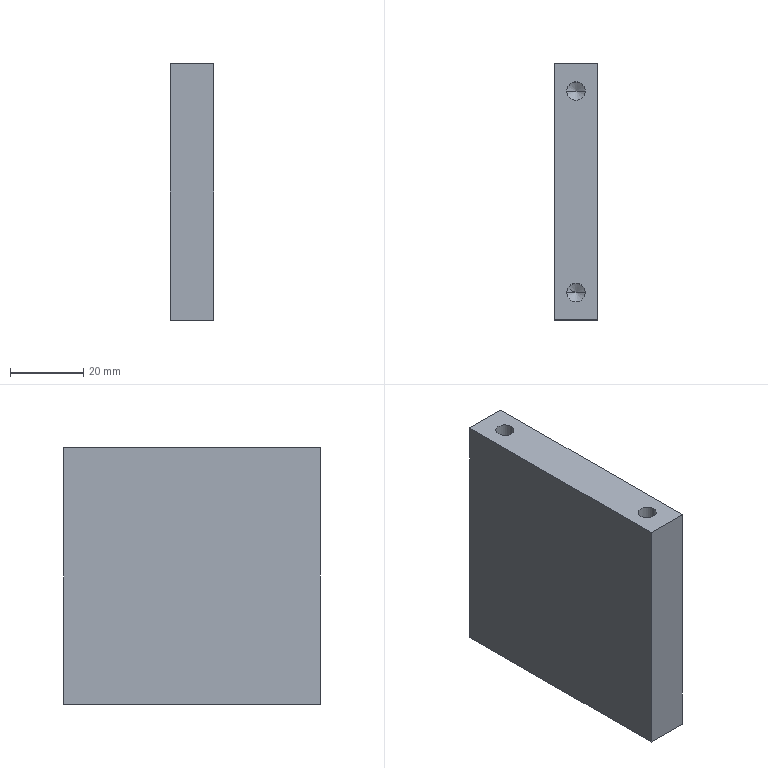Component | SolidWorks | ServoDriveMotorModule-1_WT-FLD-EJG-1212-00-020-1 | 1 solid | 22 faces | box 12 x 70 x 70 mm | volume 57583 mm3 | cylinder 8 | cone 8 | plane 6 | commonest cylinder face diameters 5 x8 | material AISI 1045 Steel, cold drawn
build123d program:
from build123d import *

# Parameters (mm, degrees)
SKETCH1_W                  = 12
SKETCH1_H                  = 70
BOSS_EXTRUDE1_DEPTH        = 35
M6_TAPPED_HOLE1_AT_2_COUNT = 2
M6_TAPPED_HOLE1_AT_2_PITCH = 55


with BuildPart() as part:
    # Sketch1 → Boss-Extrude1 (new, symmetric)
    with BuildSketch(Plane.XY):
        Rectangle(SKETCH1_W, SKETCH1_H)
    extrude(amount=BOSS_EXTRUDE1_DEPTH, both=True)

    # Sketch2 → M6 Tapped Hole1 (revolve, cut)
    with BuildSketch(Plane(origin=(0, 27.5, 35), x_dir=(0, -1, 0), z_dir=(1, 0, 0))):
        Polygon((0, 0), (0, 16.502), (2.5, 15), (2.5, 0), align=None)
    m6_tapped_hole1 = revolve(axis=Axis((0, 27.5, 41.35), (0, 0, -1)), mode=Mode.SUBTRACT)

    # M6 Tapped Hole1 at 2: M6 Tapped Hole1 ×2
    with Locations(*[(0, -i * M6_TAPPED_HOLE1_AT_2_PITCH, 0) for i in range(1, M6_TAPPED_HOLE1_AT_2_COUNT)]):
        add(m6_tapped_hole1, mode=Mode.SUBTRACT)

    # Mirror1: M6 Tapped Hole1 across plane
    add(m6_tapped_hole1.mirror(Plane.XY), mode=Mode.SUBTRACT)

    # Mirror1 copy 1 sketch → Mirror1 copy 1 (revolve, cut)
    with BuildSketch(Plane(origin=(0, -27.5, -35), x_dir=(0, -1, 0), z_dir=(1, 0, 0))):
        Polygon((0, 0), (0, -16.502), (2.5, -15), (2.5, 0), align=None)
    revolve(axis=Axis((0, -27.5, -41.35), (0, 0, -1)), mode=Mode.SUBTRACT)


solid = part.part

# Placed as in the assembly
solid = solid.moved(Location((-49, 0, 95), (0, 0, 0)))
STEP:
#1=CARTESIAN_POINT('',(-2.028,1.083,4.528));
#2=VERTEX_POINT('',#1);
#3=CARTESIAN_POINT('',(-1.831,1.083,4.528));
#4=VERTEX_POINT('',#3);
#5=CARTESIAN_POINT('',(-1.929,1.083,4.528));
#6=DIRECTION('',(0.,-0.,1.));
#7=DIRECTION('',(1.,0.,0.));
#8=AXIS2_PLACEMENT_3D('',#5,#6,#7);
#9=CIRCLE('',#8,0.09843);
#10=EDGE_CURVE('',#2,#4,#9,.T.);
#11=ORIENTED_EDGE('',*,*,#10,.F.);
#12=CARTESIAN_POINT('',(-2.028,1.083,5.118));
#13=VERTEX_POINT('',#12);
#14=CARTESIAN_POINT('',(-2.028,1.083,5.118));
#15=DIRECTION('',(0.,-0.,1.));
#16=VECTOR('',#15,39.37);
#17=LINE('',#14,#16);
#18=EDGE_CURVE('',#2,#13,#17,.T.);
#19=ORIENTED_EDGE('',*,*,#18,.T.);
#20=CARTESIAN_POINT('',(-1.831,1.083,5.118));
#21=VERTEX_POINT('',#20);
#22=CARTESIAN_POINT('',(-1.929,1.083,5.118));
#23=DIRECTION('',(0.,-0.,1.));
#24=DIRECTION('',(1.,0.,0.));
#25=AXIS2_PLACEMENT_3D('',#22,#23,#24);
#26=CIRCLE('',#25,0.09843);
#27=EDGE_CURVE('',#13,#21,#26,.T.);
#28=ORIENTED_EDGE('',*,*,#27,.T.);
#29=CARTESIAN_POINT('',(-1.831,1.083,5.118));
#30=DIRECTION('',(0.,-0.,1.));
#31=VECTOR('',#30,39.37);
#32=LINE('',#29,#31);
#33=EDGE_CURVE('',#4,#21,#32,.T.);
#34=ORIENTED_EDGE('',*,*,#33,.F.);
#35=EDGE_LOOP('',(#11,#19,#28,#34));
#36=FACE_OUTER_BOUND('',#35,.T.);
#37=CARTESIAN_POINT('',(-1.929,1.083,5.118));
#38=DIRECTION('',(0.,-0.,1.));
#39=DIRECTION('',(1.,0.,0.));
#40=AXIS2_PLACEMENT_3D('',#37,#38,#39);
#41=CYLINDRICAL_SURFACE('',#40,0.09843);
#42=ADVANCED_FACE('',(#36),#41,.F.);
#43=CARTESIAN_POINT('',(-1.929,1.083,4.468));
#44=VERTEX_POINT('',#43);
#45=CARTESIAN_POINT('',(-1.831,1.083,4.528));
#46=DIRECTION('',(0.8572,0.,0.515));
#47=VECTOR('',#46,39.37);
#48=LINE('',#45,#47);
#49=EDGE_CURVE('',#44,#4,#48,.T.);
#50=ORIENTED_EDGE('',*,*,#49,.F.);
#51=CARTESIAN_POINT('',(-2.028,1.083,4.528));
#52=DIRECTION('',(-0.8572,-0.,0.515));
#53=VECTOR('',#52,39.37);
#54=LINE('',#51,#53);
#55=EDGE_CURVE('',#44,#2,#54,.T.);
#56=ORIENTED_EDGE('',*,*,#55,.T.);
#57=ORIENTED_EDGE('',*,*,#10,.T.);
#58=EDGE_LOOP('',(#50,#56,#57));
#59=FACE_OUTER_BOUND('',#58,.T.);
#60=CARTESIAN_POINT('',(-1.929,1.083,4.528));
#61=DIRECTION('',(0.,-0.,1.));
#62=DIRECTION('',(1.,0.,0.));
#63=AXIS2_PLACEMENT_3D('',#60,#61,#62);
#64=CONICAL_SURFACE('',#63,0.09843,1.03);
#65=ADVANCED_FACE('',(#59),#64,.F.);
#66=CARTESIAN_POINT('',(-2.028,-1.083,4.528));
#67=VERTEX_POINT('',#66);
#68=CARTESIAN_POINT('',(-1.831,-1.083,4.528));
#69=VERTEX_POINT('',#68);
#70=CARTESIAN_POINT('',(-1.929,-1.083,4.528));
#71=DIRECTION('',(0.,-0.,1.));
#72=DIRECTION('',(1.,0.,0.));
#73=AXIS2_PLACEMENT_3D('',#70,#71,#72);
#74=CIRCLE('',#73,0.09843);
#75=EDGE_CURVE('',#67,#69,#74,.T.);
#76=ORIENTED_EDGE('',*,*,#75,.F.);
#77=CARTESIAN_POINT('',(-2.028,-1.083,5.118));
#78=VERTEX_POINT('',#77);
#79=CARTESIAN_POINT('',(-2.028,-1.083,5.118));
#80=DIRECTION('',(0.,-0.,1.));
#81=VECTOR('',#80,39.37);
#82=LINE('',#79,#81);
#83=EDGE_CURVE('',#67,#78,#82,.T.);
#84=ORIENTED_EDGE('',*,*,#83,.T.);
#85=CARTESIAN_POINT('',(-1.831,-1.083,5.118));
#86=VERTEX_POINT('',#85);
#87=CARTESIAN_POINT('',(-1.929,-1.083,5.118));
#88=DIRECTION('',(0.,-0.,1.));
#89=DIRECTION('',(1.,0.,0.));
#90=AXIS2_PLACEMENT_3D('',#87,#88,#89);
#91=CIRCLE('',#90,0.09843);
#92=EDGE_CURVE('',#78,#86,#91,.T.);
#93=ORIENTED_EDGE('',*,*,#92,.T.);
#94=CARTESIAN_POINT('',(-1.831,-1.083,5.118));
#95=DIRECTION('',(0.,-0.,1.));
#96=VECTOR('',#95,39.37);
#97=LINE('',#94,#96);
#98=EDGE_CURVE('',#69,#86,#97,.T.);
#99=ORIENTED_EDGE('',*,*,#98,.F.);
#100=EDGE_LOOP('',(#76,#84,#93,#99));
#101=FACE_OUTER_BOUND('',#100,.T.);
#102=CARTESIAN_POINT('',(-1.929,-1.083,5.118));
#103=DIRECTION('',(0.,-0.,1.));
#104=DIRECTION('',(1.,0.,0.));
#105=AXIS2_PLACEMENT_3D('',#102,#103,#104);
#106=CYLINDRICAL_SURFACE('',#105,0.09843);
#107=ADVANCED_FACE('',(#101),#106,.F.);
#108=CARTESIAN_POINT('',(-1.929,-1.083,4.468));
#109=VERTEX_POINT('',#108);
#110=CARTESIAN_POINT('',(-1.831,-1.083,4.528));
#111=DIRECTION('',(0.8572,0.,0.515));
#112=VECTOR('',#111,39.37);
#113=LINE('',#110,#112);
#114=EDGE_CURVE('',#109,#69,#113,.T.);
#115=ORIENTED_EDGE('',*,*,#114,.F.);
#116=CARTESIAN_POINT('',(-2.028,-1.083,4.528));
#117=DIRECTION('',(-0.8572,-0.,0.515));
#118=VECTOR('',#117,39.37);
#119=LINE('',#116,#118);
#120=EDGE_CURVE('',#109,#67,#119,.T.);
#121=ORIENTED_EDGE('',*,*,#120,.T.);
#122=ORIENTED_EDGE('',*,*,#75,.T.);
#123=EDGE_LOOP('',(#115,#121,#122));
#124=FACE_OUTER_BOUND('',#123,.T.);
#125=CARTESIAN_POINT('',(-1.929,-1.083,4.528));
#126=DIRECTION('',(0.,-0.,1.));
#127=DIRECTION('',(1.,0.,0.));
#128=AXIS2_PLACEMENT_3D('',#125,#126,#127);
#129=CONICAL_SURFACE('',#128,0.09843,1.03);
#130=ADVANCED_FACE('',(#124),#129,.F.);
#131=CARTESIAN_POINT('',(-1.831,1.083,2.953));
#132=VERTEX_POINT('',#131);
#133=CARTESIAN_POINT('',(-2.028,1.083,2.953));
#134=VERTEX_POINT('',#133);
#135=CARTESIAN_POINT('',(-1.929,1.083,2.953));
#136=DIRECTION('',(-0.,0.,-1.));
#137=DIRECTION('',(-1.,-0.,0.));
#138=AXIS2_PLACEMENT_3D('',#135,#136,#137);
#139=CIRCLE('',#138,0.09843);
#140=EDGE_CURVE('',#132,#134,#139,.T.);
#141=ORIENTED_EDGE('',*,*,#140,.F.);
#142=CARTESIAN_POINT('',(-1.831,1.083,2.362));
#143=VERTEX_POINT('',#142);
#144=CARTESIAN_POINT('',(-1.831,1.083,2.362));
#145=DIRECTION('',(-0.,0.,-1.));
#146=VECTOR('',#145,39.37);
#147=LINE('',#144,#146);
#148=EDGE_CURVE('',#132,#143,#147,.T.);
#149=ORIENTED_EDGE('',*,*,#148,.T.);
#150=CARTESIAN_POINT('',(-2.028,1.083,2.362));
#151=VERTEX_POINT('',#150);
#152=CARTESIAN_POINT('',(-1.929,1.083,2.362));
#153=DIRECTION('',(-0.,0.,-1.));
#154=DIRECTION('',(-1.,-0.,0.));
#155=AXIS2_PLACEMENT_3D('',#152,#153,#154);
#156=CIRCLE('',#155,0.09843);
#157=EDGE_CURVE('',#143,#151,#156,.T.);
#158=ORIENTED_EDGE('',*,*,#157,.T.);
#159=CARTESIAN_POINT('',(-2.028,1.083,2.362));
#160=DIRECTION('',(-0.,0.,-1.));
#161=VECTOR('',#160,39.37);
#162=LINE('',#159,#161);
#163=EDGE_CURVE('',#134,#151,#162,.T.);
#164=ORIENTED_EDGE('',*,*,#163,.F.);
#165=EDGE_LOOP('',(#141,#149,#158,#164));
#166=FACE_OUTER_BOUND('',#165,.T.);
#167=CARTESIAN_POINT('',(-1.929,1.083,2.362));
#168=DIRECTION('',(-0.,0.,-1.));
#169=DIRECTION('',(-1.,-0.,0.));
#170=AXIS2_PLACEMENT_3D('',#167,#168,#169);
#171=CYLINDRICAL_SURFACE('',#170,0.09843);
#172=ADVANCED_FACE('',(#166),#171,.F.);
#173=CARTESIAN_POINT('',(-1.929,1.083,3.012));
#174=VERTEX_POINT('',#173);
#175=CARTESIAN_POINT('',(-2.028,1.083,2.953));
#176=DIRECTION('',(-0.8572,-0.,-0.515));
#177=VECTOR('',#176,39.37);
#178=LINE('',#175,#177);
#179=EDGE_CURVE('',#174,#134,#178,.T.);
#180=ORIENTED_EDGE('',*,*,#179,.F.);
#181=CARTESIAN_POINT('',(-1.831,1.083,2.953));
#182=DIRECTION('',(0.8572,0.,-0.515));
#183=VECTOR('',#182,39.37);
#184=LINE('',#181,#183);
#185=EDGE_CURVE('',#174,#132,#184,.T.);
#186=ORIENTED_EDGE('',*,*,#185,.T.);
#187=ORIENTED_EDGE('',*,*,#140,.T.);
#188=EDGE_LOOP('',(#180,#186,#187));
#189=FACE_OUTER_BOUND('',#188,.T.);
#190=CARTESIAN_POINT('',(-1.929,1.083,2.953));
#191=DIRECTION('',(-0.,0.,-1.));
#192=DIRECTION('',(-1.,-0.,0.));
#193=AXIS2_PLACEMENT_3D('',#190,#191,#192);
#194=CONICAL_SURFACE('',#193,0.09843,1.03);
#195=ADVANCED_FACE('',(#189),#194,.F.);
#196=CARTESIAN_POINT('',(-1.831,-1.083,2.953));
#197=VERTEX_POINT('',#196);
#198=CARTESIAN_POINT('',(-2.028,-1.083,2.953));
#199=VERTEX_POINT('',#198);
#200=CARTESIAN_POINT('',(-1.929,-1.083,2.953));
#201=DIRECTION('',(-0.,0.,-1.));
#202=DIRECTION('',(-1.,-0.,0.));
#203=AXIS2_PLACEMENT_3D('',#200,#201,#202);
#204=CIRCLE('',#203,0.09843);
#205=EDGE_CURVE('',#197,#199,#204,.T.);
#206=ORIENTED_EDGE('',*,*,#205,.F.);
#207=CARTESIAN_POINT('',(-1.831,-1.083,2.362));
#208=VERTEX_POINT('',#207);
#209=CARTESIAN_POINT('',(-1.831,-1.083,2.362));
#210=DIRECTION('',(-0.,0.,-1.));
#211=VECTOR('',#210,39.37);
#212=LINE('',#209,#211);
#213=EDGE_CURVE('',#197,#208,#212,.T.);
#214=ORIENTED_EDGE('',*,*,#213,.T.);
#215=CARTESIAN_POINT('',(-2.028,-1.083,2.362));
#216=VERTEX_POINT('',#215);
#217=CARTESIAN_POINT('',(-1.929,-1.083,2.362));
#218=DIRECTION('',(-0.,0.,-1.));
#219=DIRECTION('',(-1.,-0.,0.));
#220=AXIS2_PLACEMENT_3D('',#217,#218,#219);
#221=CIRCLE('',#220,0.09843);
#222=EDGE_CURVE('',#208,#216,#221,.T.);
#223=ORIENTED_EDGE('',*,*,#222,.T.);
#224=CARTESIAN_POINT('',(-2.028,-1.083,2.362));
#225=DIRECTION('',(-0.,0.,-1.));
#226=VECTOR('',#225,39.37);
#227=LINE('',#224,#226);
#228=EDGE_CURVE('',#199,#216,#227,.T.);
#229=ORIENTED_EDGE('',*,*,#228,.F.);
#230=EDGE_LOOP('',(#206,#214,#223,#229));
#231=FACE_OUTER_BOUND('',#230,.T.);
#232=CARTESIAN_POINT('',(-1.929,-1.083,2.362));
#233=DIRECTION('',(-0.,0.,-1.));
#234=DIRECTION('',(-1.,-0.,0.));
#235=AXIS2_PLACEMENT_3D('',#232,#233,#234);
#236=CYLINDRICAL_SURFACE('',#235,0.09843);
#237=ADVANCED_FACE('',(#231),#236,.F.);
#238=CARTESIAN_POINT('',(-1.929,-1.083,3.012));
#239=VERTEX_POINT('',#238);
#240=CARTESIAN_POINT('',(-2.028,-1.083,2.953));
#241=DIRECTION('',(-0.8572,-0.,-0.515));
#242=VECTOR('',#241,39.37);
#243=LINE('',#240,#242);
#244=EDGE_CURVE('',#239,#199,#243,.T.);
#245=ORIENTED_EDGE('',*,*,#244,.F.);
#246=CARTESIAN_POINT('',(-1.831,-1.083,2.953));
#247=DIRECTION('',(0.8572,0.,-0.515));
#248=VECTOR('',#247,39.37);
#249=LINE('',#246,#248);
#250=EDGE_CURVE('',#239,#197,#249,.T.);
#251=ORIENTED_EDGE('',*,*,#250,.T.);
#252=ORIENTED_EDGE('',*,*,#205,.T.);
#253=EDGE_LOOP('',(#245,#251,#252));
#254=FACE_OUTER_BOUND('',#253,.T.);
#255=CARTESIAN_POINT('',(-1.929,-1.083,2.953));
#256=DIRECTION('',(-0.,0.,-1.));
#257=DIRECTION('',(-1.,-0.,0.));
#258=AXIS2_PLACEMENT_3D('',#255,#256,#257);
#259=CONICAL_SURFACE('',#258,0.09843,1.03);
#260=ADVANCED_FACE('',(#254),#259,.F.);
#261=CARTESIAN_POINT('',(-2.165,-1.378,5.118));
#262=VERTEX_POINT('',#261);
#263=CARTESIAN_POINT('',(-2.165,1.378,5.118));
#264=VERTEX_POINT('',#263);
#265=CARTESIAN_POINT('',(-2.165,-1.378,5.118));
#266=DIRECTION('',(-0.,1.,0.));
#267=VECTOR('',#266,39.37);
#268=LINE('',#265,#267);
#269=EDGE_CURVE('',#262,#264,#268,.T.);
#270=ORIENTED_EDGE('',*,*,#269,.T.);
#271=CARTESIAN_POINT('',(-2.165,1.378,2.362));
#272=VERTEX_POINT('',#271);
#273=CARTESIAN_POINT('',(-2.165,1.378,2.362));
#274=DIRECTION('',(0.,-0.,1.));
#275=VECTOR('',#274,39.37);
#276=LINE('',#273,#275);
#277=EDGE_CURVE('',#272,#264,#276,.T.);
#278=ORIENTED_EDGE('',*,*,#277,.F.);
#279=CARTESIAN_POINT('',(-2.165,-1.378,2.362));
#280=VERTEX_POINT('',#279);
#281=CARTESIAN_POINT('',(-2.165,-1.378,2.362));
#282=DIRECTION('',(-0.,1.,0.));
#283=VECTOR('',#282,39.37);
#284=LINE('',#281,#283);
#285=EDGE_CURVE('',#280,#272,#284,.T.);
#286=ORIENTED_EDGE('',*,*,#285,.F.);
#287=CARTESIAN_POINT('',(-2.165,-1.378,2.362));
#288=DIRECTION('',(0.,-0.,1.));
#289=VECTOR('',#288,39.37);
#290=LINE('',#287,#289);
#291=EDGE_CURVE('',#280,#262,#290,.T.);
#292=ORIENTED_EDGE('',*,*,#291,.T.);
#293=EDGE_LOOP('',(#270,#278,#286,#292));
#294=FACE_OUTER_BOUND('',#293,.T.);
#295=CARTESIAN_POINT('',(-2.165,-1.378,2.362));
#296=DIRECTION('',(1.,0.,-0.));
#297=DIRECTION('',(-0.,0.,-1.));
#298=AXIS2_PLACEMENT_3D('',#295,#296,#297);
#299=PLANE('',#298);
#300=ADVANCED_FACE('',(#294),#299,.F.);
#301=CARTESIAN_POINT('',(-1.693,1.378,5.118));
#302=VERTEX_POINT('',#301);
#303=CARTESIAN_POINT('',(-1.693,1.378,5.118));
#304=DIRECTION('',(1.,0.,-0.));
#305=VECTOR('',#304,39.37);
#306=LINE('',#303,#305);
#307=EDGE_CURVE('',#264,#302,#306,.T.);
#308=ORIENTED_EDGE('',*,*,#307,.T.);
#309=CARTESIAN_POINT('',(-1.693,1.378,2.362));
#310=VERTEX_POINT('',#309);
#311=CARTESIAN_POINT('',(-1.693,1.378,2.362));
#312=DIRECTION('',(0.,-0.,1.));
#313=VECTOR('',#312,39.37);
#314=LINE('',#311,#313);
#315=EDGE_CURVE('',#310,#302,#314,.T.);
#316=ORIENTED_EDGE('',*,*,#315,.F.);
#317=CARTESIAN_POINT('',(-1.693,1.378,2.362));
#318=DIRECTION('',(1.,0.,-0.));
#319=VECTOR('',#318,39.37);
#320=LINE('',#317,#319);
#321=EDGE_CURVE('',#272,#310,#320,.T.);
#322=ORIENTED_EDGE('',*,*,#321,.F.);
#323=ORIENTED_EDGE('',*,*,#277,.T.);
#324=EDGE_LOOP('',(#308,#316,#322,#323));
#325=FACE_OUTER_BOUND('',#324,.T.);
#326=CARTESIAN_POINT('',(-1.693,1.378,2.362));
#327=DIRECTION('',(0.,-1.,-0.));
#328=DIRECTION('',(0.,-0.,1.));
#329=AXIS2_PLACEMENT_3D('',#326,#327,#328);
#330=PLANE('',#329);
#331=ADVANCED_FACE('',(#325),#330,.F.);
#332=CARTESIAN_POINT('',(-1.693,-1.378,5.118));
#333=VERTEX_POINT('',#332);
#334=CARTESIAN_POINT('',(-1.693,-1.378,5.118));
#335=DIRECTION('',(0.,-1.,-0.));
#336=VECTOR('',#335,39.37);
#337=LINE('',#334,#336);
#338=EDGE_CURVE('',#302,#333,#337,.T.);
#339=ORIENTED_EDGE('',*,*,#338,.T.);
#340=CARTESIAN_POINT('',(-1.693,-1.378,2.362));
#341=VERTEX_POINT('',#340);
#342=CARTESIAN_POINT('',(-1.693,-1.378,2.362));
#343=DIRECTION('',(0.,-0.,1.));
#344=VECTOR('',#343,39.37);
#345=LINE('',#342,#344);
#346=EDGE_CURVE('',#341,#333,#345,.T.);
#347=ORIENTED_EDGE('',*,*,#346,.F.);
#348=CARTESIAN_POINT('',(-1.693,-1.378,2.362));
#349=DIRECTION('',(0.,-1.,-0.));
#350=VECTOR('',#349,39.37);
#351=LINE('',#348,#350);
#352=EDGE_CURVE('',#310,#341,#351,.T.);
#353=ORIENTED_EDGE('',*,*,#352,.F.);
#354=ORIENTED_EDGE('',*,*,#315,.T.);
#355=EDGE_LOOP('',(#339,#347,#353,#354));
#356=FACE_OUTER_BOUND('',#355,.T.);
#357=CARTESIAN_POINT('',(-1.693,-1.378,2.362));
#358=DIRECTION('',(-1.,-0.,0.));
#359=DIRECTION('',(0.,-0.,1.));
#360=AXIS2_PLACEMENT_3D('',#357,#358,#359);
#361=PLANE('',#360);
#362=ADVANCED_FACE('',(#356),#361,.F.);
#363=CARTESIAN_POINT('',(-1.693,-1.378,5.118));
#364=DIRECTION('',(-1.,-0.,0.));
#365=VECTOR('',#364,39.37);
#366=LINE('',#363,#365);
#367=EDGE_CURVE('',#333,#262,#366,.T.);
#368=ORIENTED_EDGE('',*,*,#367,.T.);
#369=ORIENTED_EDGE('',*,*,#291,.F.);
#370=CARTESIAN_POINT('',(-1.693,-1.378,2.362));
#371=DIRECTION('',(-1.,-0.,0.));
#372=VECTOR('',#371,39.37);
#373=LINE('',#370,#372);
#374=EDGE_CURVE('',#341,#280,#373,.T.);
#375=ORIENTED_EDGE('',*,*,#374,.F.);
#376=ORIENTED_EDGE('',*,*,#346,.T.);
#377=EDGE_LOOP('',(#368,#369,#375,#376));
#378=FACE_OUTER_BOUND('',#377,.T.);
#379=CARTESIAN_POINT('',(-1.693,-1.378,2.362));
#380=DIRECTION('',(-0.,1.,0.));
#381=DIRECTION('',(-0.,0.,-1.));
#382=AXIS2_PLACEMENT_3D('',#379,#380,#381);
#383=PLANE('',#382);
#384=ADVANCED_FACE('',(#378),#383,.F.);
#385=CARTESIAN_POINT('',(-1.929,1.083,2.362));
#386=DIRECTION('',(-0.,0.,-1.));
#387=DIRECTION('',(-1.,-0.,0.));
#388=AXIS2_PLACEMENT_3D('',#385,#386,#387);
#389=CIRCLE('',#388,0.09843);
#390=EDGE_CURVE('',#151,#143,#389,.T.);
#391=ORIENTED_EDGE('',*,*,#390,.F.);
#392=ORIENTED_EDGE('',*,*,#157,.F.);
#393=EDGE_LOOP('',(#391,#392));
#394=FACE_BOUND('',#393,.T.);
#395=CARTESIAN_POINT('',(-1.929,-1.083,2.362));
#396=DIRECTION('',(-0.,0.,-1.));
#397=DIRECTION('',(-1.,-0.,0.));
#398=AXIS2_PLACEMENT_3D('',#395,#396,#397);
#399=CIRCLE('',#398,0.09843);
#400=EDGE_CURVE('',#216,#208,#399,.T.);
#401=ORIENTED_EDGE('',*,*,#400,.F.);
#402=ORIENTED_EDGE('',*,*,#222,.F.);
#403=EDGE_LOOP('',(#401,#402));
#404=FACE_BOUND('',#403,.T.);
#405=ORIENTED_EDGE('',*,*,#285,.T.);
#406=ORIENTED_EDGE('',*,*,#321,.T.);
#407=ORIENTED_EDGE('',*,*,#352,.T.);
#408=ORIENTED_EDGE('',*,*,#374,.T.);
#409=EDGE_LOOP('',(#405,#406,#407,#408));
#410=FACE_OUTER_BOUND('',#409,.T.);
#411=CARTESIAN_POINT('',(-1.929,-0.,2.362));
#412=DIRECTION('',(0.,-0.,1.));
#413=DIRECTION('',(1.,0.,-0.));
#414=AXIS2_PLACEMENT_3D('',#411,#412,#413);
#415=PLANE('',#414);
#416=ADVANCED_FACE('',(#394,#404,#410),#415,.F.);
#417=CARTESIAN_POINT('',(-1.929,1.083,5.118));
#418=DIRECTION('',(0.,-0.,1.));
#419=DIRECTION('',(1.,0.,0.));
#420=AXIS2_PLACEMENT_3D('',#417,#418,#419);
#421=CIRCLE('',#420,0.09843);
#422=EDGE_CURVE('',#21,#13,#421,.T.);
#423=ORIENTED_EDGE('',*,*,#422,.F.);
#424=ORIENTED_EDGE('',*,*,#27,.F.);
#425=EDGE_LOOP('',(#423,#424));
#426=FACE_BOUND('',#425,.T.);
#427=CARTESIAN_POINT('',(-1.929,-1.083,5.118));
#428=DIRECTION('',(0.,-0.,1.));
#429=DIRECTION('',(1.,0.,0.));
#430=AXIS2_PLACEMENT_3D('',#427,#428,#429);
#431=CIRCLE('',#430,0.09843);
#432=EDGE_CURVE('',#86,#78,#431,.T.);
#433=ORIENTED_EDGE('',*,*,#432,.F.);
#434=ORIENTED_EDGE('',*,*,#92,.F.);
#435=EDGE_LOOP('',(#433,#434));
#436=FACE_BOUND('',#435,.T.);
#437=ORIENTED_EDGE('',*,*,#269,.F.);
#438=ORIENTED_EDGE('',*,*,#367,.F.);
#439=ORIENTED_EDGE('',*,*,#338,.F.);
#440=ORIENTED_EDGE('',*,*,#307,.F.);
#441=EDGE_LOOP('',(#437,#438,#439,#440));
#442=FACE_OUTER_BOUND('',#441,.T.);
#443=CARTESIAN_POINT('',(-1.929,-0.,5.118));
#444=DIRECTION('',(0.,-0.,1.));
#445=DIRECTION('',(1.,0.,-0.));
#446=AXIS2_PLACEMENT_3D('',#443,#444,#445);
#447=PLANE('',#446);
#448=ADVANCED_FACE('',(#426,#436,#442),#447,.T.);
#449=ORIENTED_EDGE('',*,*,#250,.F.);
#450=ORIENTED_EDGE('',*,*,#244,.T.);
#451=CARTESIAN_POINT('',(-1.929,-1.083,2.953));
#452=DIRECTION('',(-0.,0.,-1.));
#453=DIRECTION('',(-1.,-0.,0.));
#454=AXIS2_PLACEMENT_3D('',#451,#452,#453);
#455=CIRCLE('',#454,0.09843);
#456=EDGE_CURVE('',#199,#197,#455,.T.);
#457=ORIENTED_EDGE('',*,*,#456,.T.);
#458=EDGE_LOOP('',(#449,#450,#457));
#459=FACE_OUTER_BOUND('',#458,.T.);
#460=CARTESIAN_POINT('',(-1.929,-1.083,2.953));
#461=DIRECTION('',(-0.,0.,-1.));
#462=DIRECTION('',(-1.,-0.,0.));
#463=AXIS2_PLACEMENT_3D('',#460,#461,#462);
#464=CONICAL_SURFACE('',#463,0.09843,1.03);
#465=ADVANCED_FACE('',(#459),#464,.F.);
#466=ORIENTED_EDGE('',*,*,#213,.F.);
#467=ORIENTED_EDGE('',*,*,#456,.F.);
#468=ORIENTED_EDGE('',*,*,#228,.T.);
#469=ORIENTED_EDGE('',*,*,#400,.T.);
#470=EDGE_LOOP('',(#466,#467,#468,#469));
#471=FACE_OUTER_BOUND('',#470,.T.);
#472=CARTESIAN_POINT('',(-1.929,-1.083,2.362));
#473=DIRECTION('',(-0.,0.,-1.));
#474=DIRECTION('',(-1.,-0.,0.));
#475=AXIS2_PLACEMENT_3D('',#472,#473,#474);
#476=CYLINDRICAL_SURFACE('',#475,0.09843);
#477=ADVANCED_FACE('',(#471),#476,.F.);
#478=ORIENTED_EDGE('',*,*,#185,.F.);
#479=ORIENTED_EDGE('',*,*,#179,.T.);
#480=CARTESIAN_POINT('',(-1.929,1.083,2.953));
#481=DIRECTION('',(-0.,0.,-1.));
#482=DIRECTION('',(-1.,-0.,0.));
#483=AXIS2_PLACEMENT_3D('',#480,#481,#482);
#484=CIRCLE('',#483,0.09843);
#485=EDGE_CURVE('',#134,#132,#484,.T.);
#486=ORIENTED_EDGE('',*,*,#485,.T.);
#487=EDGE_LOOP('',(#478,#479,#486));
#488=FACE_OUTER_BOUND('',#487,.T.);
#489=CARTESIAN_POINT('',(-1.929,1.083,2.953));
#490=DIRECTION('',(-0.,0.,-1.));
#491=DIRECTION('',(-1.,-0.,0.));
#492=AXIS2_PLACEMENT_3D('',#489,#490,#491);
#493=CONICAL_SURFACE('',#492,0.09843,1.03);
#494=ADVANCED_FACE('',(#488),#493,.F.);
#495=ORIENTED_EDGE('',*,*,#148,.F.);
#496=ORIENTED_EDGE('',*,*,#485,.F.);
#497=ORIENTED_EDGE('',*,*,#163,.T.);
#498=ORIENTED_EDGE('',*,*,#390,.T.);
#499=EDGE_LOOP('',(#495,#496,#497,#498));
#500=FACE_OUTER_BOUND('',#499,.T.);
#501=CARTESIAN_POINT('',(-1.929,1.083,2.362));
#502=DIRECTION('',(-0.,0.,-1.));
#503=DIRECTION('',(-1.,-0.,0.));
#504=AXIS2_PLACEMENT_3D('',#501,#502,#503);
#505=CYLINDRICAL_SURFACE('',#504,0.09843);
#506=ADVANCED_FACE('',(#500),#505,.F.);
#507=ORIENTED_EDGE('',*,*,#120,.F.);
#508=ORIENTED_EDGE('',*,*,#114,.T.);
#509=CARTESIAN_POINT('',(-1.929,-1.083,4.528));
#510=DIRECTION('',(0.,-0.,1.));
#511=DIRECTION('',(1.,0.,0.));
#512=AXIS2_PLACEMENT_3D('',#509,#510,#511);
#513=CIRCLE('',#512,0.09843);
#514=EDGE_CURVE('',#69,#67,#513,.T.);
#515=ORIENTED_EDGE('',*,*,#514,.T.);
#516=EDGE_LOOP('',(#507,#508,#515));
#517=FACE_OUTER_BOUND('',#516,.T.);
#518=CARTESIAN_POINT('',(-1.929,-1.083,4.528));
#519=DIRECTION('',(0.,-0.,1.));
#520=DIRECTION('',(1.,0.,0.));
#521=AXIS2_PLACEMENT_3D('',#518,#519,#520);
#522=CONICAL_SURFACE('',#521,0.09843,1.03);
#523=ADVANCED_FACE('',(#517),#522,.F.);
#524=ORIENTED_EDGE('',*,*,#83,.F.);
#525=ORIENTED_EDGE('',*,*,#514,.F.);
#526=ORIENTED_EDGE('',*,*,#98,.T.);
#527=ORIENTED_EDGE('',*,*,#432,.T.);
#528=EDGE_LOOP('',(#524,#525,#526,#527));
#529=FACE_OUTER_BOUND('',#528,.T.);
#530=CARTESIAN_POINT('',(-1.929,-1.083,5.118));
#531=DIRECTION('',(0.,-0.,1.));
#532=DIRECTION('',(1.,0.,0.));
#533=AXIS2_PLACEMENT_3D('',#530,#531,#532);
#534=CYLINDRICAL_SURFACE('',#533,0.09843);
#535=ADVANCED_FACE('',(#529),#534,.F.);
#536=ORIENTED_EDGE('',*,*,#55,.F.);
#537=ORIENTED_EDGE('',*,*,#49,.T.);
#538=CARTESIAN_POINT('',(-1.929,1.083,4.528));
#539=DIRECTION('',(0.,-0.,1.));
#540=DIRECTION('',(1.,0.,0.));
#541=AXIS2_PLACEMENT_3D('',#538,#539,#540);
#542=CIRCLE('',#541,0.09843);
#543=EDGE_CURVE('',#4,#2,#542,.T.);
#544=ORIENTED_EDGE('',*,*,#543,.T.);
#545=EDGE_LOOP('',(#536,#537,#544));
#546=FACE_OUTER_BOUND('',#545,.T.);
#547=CARTESIAN_POINT('',(-1.929,1.083,4.528));
#548=DIRECTION('',(0.,-0.,1.));
#549=DIRECTION('',(1.,0.,0.));
#550=AXIS2_PLACEMENT_3D('',#547,#548,#549);
#551=CONICAL_SURFACE('',#550,0.09843,1.03);
#552=ADVANCED_FACE('',(#546),#551,.F.);
#553=ORIENTED_EDGE('',*,*,#18,.F.);
#554=ORIENTED_EDGE('',*,*,#543,.F.);
#555=ORIENTED_EDGE('',*,*,#33,.T.);
#556=ORIENTED_EDGE('',*,*,#422,.T.);
#557=EDGE_LOOP('',(#553,#554,#555,#556));
#558=FACE_OUTER_BOUND('',#557,.T.);
#559=CARTESIAN_POINT('',(-1.929,1.083,5.118));
#560=DIRECTION('',(0.,-0.,1.));
#561=DIRECTION('',(1.,0.,0.));
#562=AXIS2_PLACEMENT_3D('',#559,#560,#561);
#563=CYLINDRICAL_SURFACE('',#562,0.09843);
#564=ADVANCED_FACE('',(#558),#563,.F.);
#565=CLOSED_SHELL('',(#42,#65,#107,#130,#172,#195,#237,#260,#300,#331,#362,#384,#416,#448,#465,#477,#494,#506,#523,#535,#552,#564));
#566=MANIFOLD_SOLID_BREP('',#565);
#567=CARTESIAN_POINT('',(0.,0.,0.));
#568=DIRECTION('',(0.,0.,1.));
#569=DIRECTION('',(1.,0.,0.));
#570=AXIS2_PLACEMENT_3D('',#567,#568,#569);
#571=(LENGTH_UNIT()NAMED_UNIT(*)SI_UNIT($,.METRE.));
#572=LENGTH_MEASURE_WITH_UNIT(LENGTH_MEASURE(0.0254),#571);
#573=DIMENSIONAL_EXPONENTS(1.,0.,0.,0.,0.,0.,0.);
#574=(CONVERSION_BASED_UNIT('',#572)LENGTH_UNIT()NAMED_UNIT(#573));
#575=UNCERTAINTY_MEASURE_WITH_UNIT(LENGTH_MEASURE(0.00001),#574,'','');
#576=(NAMED_UNIT(*)PLANE_ANGLE_UNIT()SI_UNIT($,.RADIAN.));
#577=(NAMED_UNIT(*)SI_UNIT($,.STERADIAN.)SOLID_ANGLE_UNIT());
#578=(GEOMETRIC_REPRESENTATION_CONTEXT(3)GLOBAL_UNCERTAINTY_ASSIGNED_CONTEXT((#575))GLOBAL_UNIT_ASSIGNED_CONTEXT((#574,#576,#577))REPRESENTATION_CONTEXT('',''));
#579=ADVANCED_BREP_SHAPE_REPRESENTATION('',(#566,#570),#578);
#580=COLOUR_RGB('',0.7922,0.8196,0.9333);
#581=FILL_AREA_STYLE_COLOUR('',#580);
#582=FILL_AREA_STYLE('',(#581));
#583=SURFACE_STYLE_FILL_AREA(#582);
#584=SURFACE_SIDE_STYLE('',(#583));
#585=SURFACE_STYLE_USAGE(.BOTH.,#584);
#586=PRESENTATION_STYLE_ASSIGNMENT((#585));
#587=STYLED_ITEM('',(#586),#566);
#588=(LENGTH_UNIT()NAMED_UNIT(*)SI_UNIT($,.METRE.));
#589=LENGTH_MEASURE_WITH_UNIT(LENGTH_MEASURE(0.0254),#588);
#590=DIMENSIONAL_EXPONENTS(1.,0.,0.,0.,0.,0.,0.);
#591=(CONVERSION_BASED_UNIT('',#589)LENGTH_UNIT()NAMED_UNIT(#590));
#592=UNCERTAINTY_MEASURE_WITH_UNIT(LENGTH_MEASURE(0.00001),#591,'','');
#593=(NAMED_UNIT(*)PLANE_ANGLE_UNIT()SI_UNIT($,.RADIAN.));
#594=(NAMED_UNIT(*)SI_UNIT($,.STERADIAN.)SOLID_ANGLE_UNIT());
#595=(GEOMETRIC_REPRESENTATION_CONTEXT(3)GLOBAL_UNCERTAINTY_ASSIGNED_CONTEXT((#592))GLOBAL_UNIT_ASSIGNED_CONTEXT((#591,#593,#594))REPRESENTATION_CONTEXT('',''));
#596=MECHANICAL_DESIGN_GEOMETRIC_PRESENTATION_REPRESENTATION('',(#587),#595);
#597=PRESENTATION_LAYER_ASSIGNMENT('','',(#587));